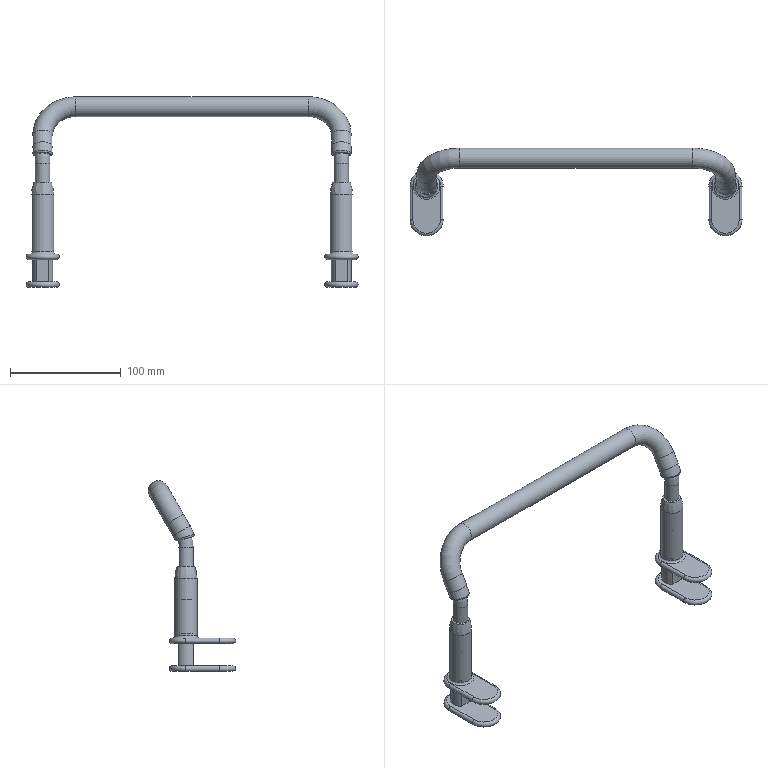Assembly | NX | mm | 6 component files | 6 solids | 92 faces | box 300 x 79 x 172.3 mm | volume 120222 mm3 | cylinder 34 | torus 26 | plane 20 | cone 8 | spline 4 | commonest cylinder face diameters 13 x10 18 x9 5 x8 10 x5 20 x2
Bill of materials:
unnamed part 1 | 2 |  | Flat oblong (stadium-shaped) base plate with rounded edges, and a solid upright post near one rounded end. The post has a chamfered top edge and at least one flat face on its side, so its cross-section is not fully round.
unnamed part 2 | 1 |  | Round rod bent into a U shape: one long straight span with a rounded bend at each end leading into a parallel leg. Each leg has an extra offset (joggle) bend, so the leg ends are displaced from the plane of the main span.
unnamed part 3 | 1 |  | Round tube bent into a U shape: one long straight span with a rounded bend at each end into short legs. The leg ends are open and hollow. In the isometric view the legs look angled rather than vertical.
unnamed part 4 | 2 |  | Flat oblong (stadium-shaped) base plate with rounded edges, and an upright hollow cylindrical post near one end. There is a fillet where the post meets the plate, and the post top is rounded. A circular bore runs down the post and appears to pass through the base.
Mates:
1. touch align | upper_mount 2 | lower_mount 2
2. distance | upper_mount 2 | lower_mount 2
3. touch align | foam_pad 1 | metal_support_rod 1
4. touch align | foam_pad 1 | metal_support_rod 1
5. touch align | metal_support_rod 1 | upper_mount 2
6. distance | metal_support_rod 1 | upper_mount 2
7. fix | assembly component
8. bond | upper_mount 2 component | assembly component
9. bond | lower_mount 2 component | assembly component
10. bond | upper_mount 1 component | assembly component
11. bond | lower_mount 1 component | assembly component
12. linear | assembly datumaxis | assembly cartesiancoordinatesystem | assembly cartesiancoordinatesystem
13. linear | assembly datumaxis | assembly cartesiancoordinatesystem | assembly cartesiancoordinatesystem